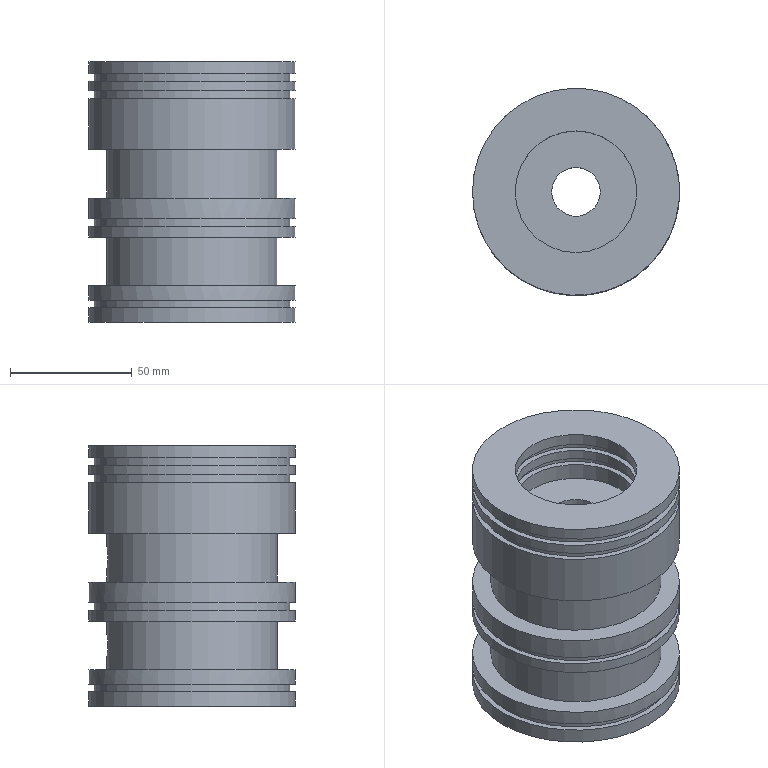Component | NX | CH3404_8-4 | 1 solid | 61 faces | volume 394985 mm3 | cylinder 31 | plane 29 | cone 1 | commonest cylinder face diameters 85 x7 80.4 x4 30 x3 20 x3 50 x3 34.6 x2 24.6 x2 54.6 x2